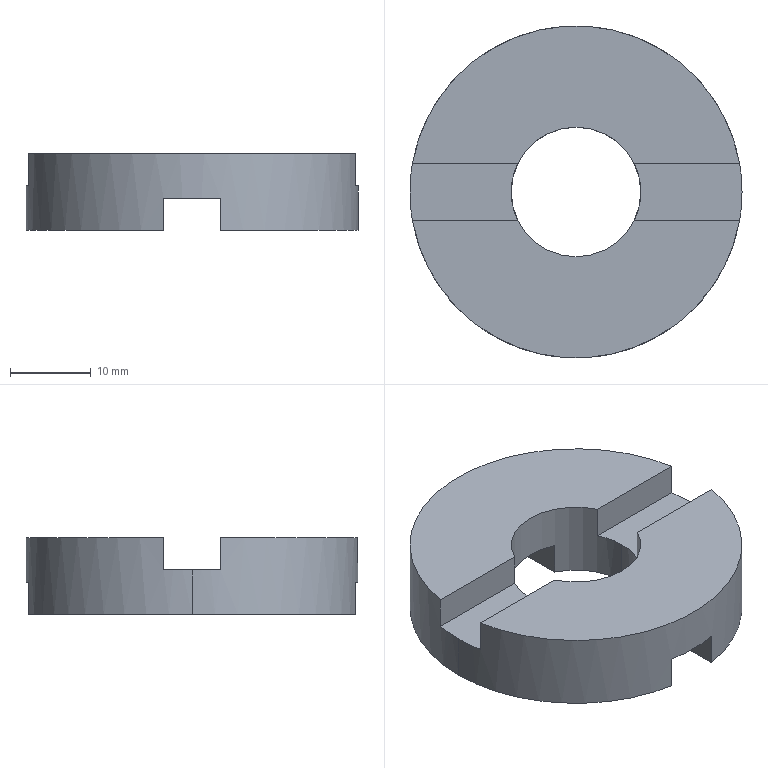Component | SolidWorks | ServoDriveMotorModule-1_MCOCGWK38_16_16-1_MCOCG_spacer38-1 | 1 solid | 20 faces | box 41 x 41 x 9.5 mm | volume 9214 mm3 | plane 16 | cylinder 4 | commonest cylinder face diameters 16 x2 41 x2 | material AISI 1045 Steel, cold drawn
build123d program:
from build123d import *

# Parameters (mm, degrees)
SKETCH1_W               = 9.5
SKETCH1_H               = 12.5
CUT_EXTRUDE1_DEPTH      = 20.5
CUT_EXTRUDE1_DEPTH_BACK = 20.5
SKETCH2_W               = 4
SKETCH2_H               = 7
CUT_EXTRUDE2_DEPTH      = 20.5
CUT_EXTRUDE2_DEPTH_BACK = 20.5
SKETCH3_W               = 4
SKETCH3_H               = 7


with BuildPart() as part:
    # Sketch1 → Revolve1 (revolve)
    with BuildSketch(Plane.XY, mode=Mode.PRIVATE) as revolve1_sk:
        with Locations((4.75, 14.25)):
            Rectangle(SKETCH1_W, SKETCH1_H)
    revolve(revolve1_sk.sketch.rotate(Axis((9.5, 0, 0), (-1, 0, 0)), 270), axis=Axis((9.5, 0, 0), (-1, 0, 0)))

    # Sketch2 → Cut-Extrude1 (cut, two sides: drawn at the far end of the back side and taken through both)
    with BuildSketch(Plane.XY.offset(-CUT_EXTRUDE1_DEPTH_BACK)):
        with Locations((2, 0)):
            Rectangle(SKETCH2_W, SKETCH2_H)
    extrude(amount=CUT_EXTRUDE1_DEPTH + CUT_EXTRUDE1_DEPTH_BACK, mode=Mode.SUBTRACT)

    # Sketch3 → Cut-Extrude2 (cut, two sides: drawn at the far end of the back side and taken through both)
    with BuildSketch(Plane(origin=(0, 0, 0), x_dir=(1, 0, 0), z_dir=(0, 1, 0)).offset(-CUT_EXTRUDE2_DEPTH_BACK)):
        with Locations((7.5, 0)):
            Rectangle(SKETCH3_W, SKETCH3_H)
    extrude(amount=CUT_EXTRUDE2_DEPTH + CUT_EXTRUDE2_DEPTH_BACK, mode=Mode.SUBTRACT)


solid = part.part

# Placed as in the assembly
solid = solid.moved(Location((0, 0, 101), (0, 90, 0)))
STEP:
#1=COLOUR_RGB('',0.7922,0.8196,0.9333);
#2=FILL_AREA_STYLE_COLOUR('',#1);
#3=FILL_AREA_STYLE('',(#2));
#4=SURFACE_STYLE_FILL_AREA(#3);
#5=SURFACE_SIDE_STYLE('',(#4));
#6=SURFACE_STYLE_USAGE(.BOTH.,#5);
#7=PRESENTATION_STYLE_ASSIGNMENT((#6));
#8=CARTESIAN_POINT('',(-0.315,0.,3.602));
#9=VERTEX_POINT('',#8);
#10=CARTESIAN_POINT('',(-0.1378,-0.2832,3.602));
#11=VERTEX_POINT('',#10);
#12=CARTESIAN_POINT('',(0.,0.,3.602));
#13=DIRECTION('',(0.,-0.,1.));
#14=DIRECTION('',(1.,0.,0.));
#15=AXIS2_PLACEMENT_3D('',#12,#13,#14);
#16=CIRCLE('',#15,0.315);
#17=EDGE_CURVE('',#9,#11,#16,.T.);
#18=ORIENTED_EDGE('',*,*,#17,.F.);
#19=CARTESIAN_POINT('',(-0.315,0.,3.819));
#20=VERTEX_POINT('',#19);
#21=CARTESIAN_POINT('',(-0.315,0.,3.602));
#22=DIRECTION('',(0.,-0.,1.));
#23=VECTOR('',#22,39.37);
#24=LINE('',#21,#23);
#25=EDGE_CURVE('',#9,#20,#24,.T.);
#26=ORIENTED_EDGE('',*,*,#25,.T.);
#27=CARTESIAN_POINT('',(-0.2832,-0.1378,3.819));
#28=VERTEX_POINT('',#27);
#29=CARTESIAN_POINT('',(0.,0.,3.819));
#30=DIRECTION('',(0.,-0.,1.));
#31=DIRECTION('',(-1.,-0.,0.));
#32=AXIS2_PLACEMENT_3D('',#29,#30,#31);
#33=CIRCLE('',#32,0.315);
#34=EDGE_CURVE('',#20,#28,#33,.T.);
#35=ORIENTED_EDGE('',*,*,#34,.T.);
#36=CARTESIAN_POINT('',(-0.2832,-0.1378,3.976));
#37=VERTEX_POINT('',#36);
#38=CARTESIAN_POINT('',(-0.2832,-0.1378,3.602));
#39=DIRECTION('',(0.,-0.,1.));
#40=VECTOR('',#39,39.37);
#41=LINE('',#38,#40);
#42=EDGE_CURVE('',#28,#37,#41,.T.);
#43=ORIENTED_EDGE('',*,*,#42,.T.);
#44=CARTESIAN_POINT('',(0.2832,-0.1378,3.976));
#45=VERTEX_POINT('',#44);
#46=CARTESIAN_POINT('',(0.,0.,3.976));
#47=DIRECTION('',(0.,-0.,1.));
#48=DIRECTION('',(1.,0.,0.));
#49=AXIS2_PLACEMENT_3D('',#46,#47,#48);
#50=CIRCLE('',#49,0.315);
#51=EDGE_CURVE('',#37,#45,#50,.T.);
#52=ORIENTED_EDGE('',*,*,#51,.T.);
#53=CARTESIAN_POINT('',(0.2832,-0.1378,3.819));
#54=VERTEX_POINT('',#53);
#55=CARTESIAN_POINT('',(0.2832,-0.1378,3.602));
#56=DIRECTION('',(-0.,0.,-1.));
#57=VECTOR('',#56,39.37);
#58=LINE('',#55,#57);
#59=EDGE_CURVE('',#45,#54,#58,.T.);
#60=ORIENTED_EDGE('',*,*,#59,.T.);
#61=CARTESIAN_POINT('',(0.315,0.,3.819));
#62=VERTEX_POINT('',#61);
#63=CARTESIAN_POINT('',(0.,0.,3.819));
#64=DIRECTION('',(0.,-0.,1.));
#65=DIRECTION('',(-1.,0.,0.));
#66=AXIS2_PLACEMENT_3D('',#63,#64,#65);
#67=CIRCLE('',#66,0.315);
#68=EDGE_CURVE('',#54,#62,#67,.T.);
#69=ORIENTED_EDGE('',*,*,#68,.T.);
#70=CARTESIAN_POINT('',(0.315,0.,3.602));
#71=VERTEX_POINT('',#70);
#72=CARTESIAN_POINT('',(0.315,0.,3.602));
#73=DIRECTION('',(0.,-0.,1.));
#74=VECTOR('',#73,39.37);
#75=LINE('',#72,#74);
#76=EDGE_CURVE('',#71,#62,#75,.T.);
#77=ORIENTED_EDGE('',*,*,#76,.F.);
#78=CARTESIAN_POINT('',(0.1378,-0.2832,3.602));
#79=VERTEX_POINT('',#78);
#80=CARTESIAN_POINT('',(0.,0.,3.602));
#81=DIRECTION('',(0.,-0.,1.));
#82=DIRECTION('',(1.,0.,0.));
#83=AXIS2_PLACEMENT_3D('',#80,#81,#82);
#84=CIRCLE('',#83,0.315);
#85=EDGE_CURVE('',#79,#71,#84,.T.);
#86=ORIENTED_EDGE('',*,*,#85,.F.);
#87=CARTESIAN_POINT('',(0.1378,-0.2832,3.76));
#88=VERTEX_POINT('',#87);
#89=CARTESIAN_POINT('',(0.1378,-0.2832,3.602));
#90=DIRECTION('',(0.,-0.,1.));
#91=VECTOR('',#90,39.37);
#92=LINE('',#89,#91);
#93=EDGE_CURVE('',#79,#88,#92,.T.);
#94=ORIENTED_EDGE('',*,*,#93,.T.);
#95=CARTESIAN_POINT('',(-0.1378,-0.2832,3.76));
#96=VERTEX_POINT('',#95);
#97=CARTESIAN_POINT('',(0.,0.,3.76));
#98=DIRECTION('',(-0.,0.,-1.));
#99=DIRECTION('',(1.,0.,0.));
#100=AXIS2_PLACEMENT_3D('',#97,#98,#99);
#101=CIRCLE('',#100,0.315);
#102=EDGE_CURVE('',#88,#96,#101,.T.);
#103=ORIENTED_EDGE('',*,*,#102,.T.);
#104=CARTESIAN_POINT('',(-0.1378,-0.2832,3.602));
#105=DIRECTION('',(-0.,0.,-1.));
#106=VECTOR('',#105,39.37);
#107=LINE('',#104,#106);
#108=EDGE_CURVE('',#96,#11,#107,.T.);
#109=ORIENTED_EDGE('',*,*,#108,.T.);
#110=EDGE_LOOP('',(#18,#26,#35,#43,#52,#60,#69,#77,#86,#94,#103,#109));
#111=FACE_OUTER_BOUND('',#110,.T.);
#112=CARTESIAN_POINT('',(0.,0.,3.602));
#113=DIRECTION('',(0.,-0.,1.));
#114=DIRECTION('',(1.,0.,0.));
#115=AXIS2_PLACEMENT_3D('',#112,#113,#114);
#116=CYLINDRICAL_SURFACE('',#115,0.315);
#117=ADVANCED_FACE('',(#111),#116,.F.);
#118=CARTESIAN_POINT('',(-0.1378,0.7952,3.602));
#119=VERTEX_POINT('',#118);
#120=CARTESIAN_POINT('',(-0.8071,-0.,3.602));
#121=VERTEX_POINT('',#120);
#122=CARTESIAN_POINT('',(0.,0.,3.602));
#123=DIRECTION('',(0.,-0.,1.));
#124=DIRECTION('',(1.,0.,0.));
#125=AXIS2_PLACEMENT_3D('',#122,#123,#124);
#126=CIRCLE('',#125,0.8071);
#127=EDGE_CURVE('',#119,#121,#126,.T.);
#128=ORIENTED_EDGE('',*,*,#127,.T.);
#129=CARTESIAN_POINT('',(-0.8071,-0.,3.819));
#130=VERTEX_POINT('',#129);
#131=CARTESIAN_POINT('',(-0.8071,-0.,3.602));
#132=DIRECTION('',(0.,-0.,1.));
#133=VECTOR('',#132,39.37);
#134=LINE('',#131,#133);
#135=EDGE_CURVE('',#121,#130,#134,.T.);
#136=ORIENTED_EDGE('',*,*,#135,.T.);
#137=CARTESIAN_POINT('',(-0.7952,0.1378,3.819));
#138=VERTEX_POINT('',#137);
#139=CARTESIAN_POINT('',(0.,0.,3.819));
#140=DIRECTION('',(-0.,0.,-1.));
#141=DIRECTION('',(-1.,-0.,0.));
#142=AXIS2_PLACEMENT_3D('',#139,#140,#141);
#143=CIRCLE('',#142,0.8071);
#144=EDGE_CURVE('',#130,#138,#143,.T.);
#145=ORIENTED_EDGE('',*,*,#144,.T.);
#146=CARTESIAN_POINT('',(-0.7952,0.1378,3.976));
#147=VERTEX_POINT('',#146);
#148=CARTESIAN_POINT('',(-0.7952,0.1378,3.602));
#149=DIRECTION('',(0.,-0.,1.));
#150=VECTOR('',#149,39.37);
#151=LINE('',#148,#150);
#152=EDGE_CURVE('',#138,#147,#151,.T.);
#153=ORIENTED_EDGE('',*,*,#152,.T.);
#154=CARTESIAN_POINT('',(0.7952,0.1378,3.976));
#155=VERTEX_POINT('',#154);
#156=CARTESIAN_POINT('',(0.,0.,3.976));
#157=DIRECTION('',(0.,-0.,1.));
#158=DIRECTION('',(1.,0.,0.));
#159=AXIS2_PLACEMENT_3D('',#156,#157,#158);
#160=CIRCLE('',#159,0.8071);
#161=EDGE_CURVE('',#155,#147,#160,.T.);
#162=ORIENTED_EDGE('',*,*,#161,.F.);
#163=CARTESIAN_POINT('',(0.7952,0.1378,3.819));
#164=VERTEX_POINT('',#163);
#165=CARTESIAN_POINT('',(0.7952,0.1378,3.602));
#166=DIRECTION('',(-0.,0.,-1.));
#167=VECTOR('',#166,39.37);
#168=LINE('',#165,#167);
#169=EDGE_CURVE('',#155,#164,#168,.T.);
#170=ORIENTED_EDGE('',*,*,#169,.T.);
#171=CARTESIAN_POINT('',(0.8071,0.,3.819));
#172=VERTEX_POINT('',#171);
#173=CARTESIAN_POINT('',(0.,0.,3.819));
#174=DIRECTION('',(-0.,0.,-1.));
#175=DIRECTION('',(-1.,-0.,0.));
#176=AXIS2_PLACEMENT_3D('',#173,#174,#175);
#177=CIRCLE('',#176,0.8071);
#178=EDGE_CURVE('',#164,#172,#177,.T.);
#179=ORIENTED_EDGE('',*,*,#178,.T.);
#180=CARTESIAN_POINT('',(0.8071,0.,3.602));
#181=VERTEX_POINT('',#180);
#182=CARTESIAN_POINT('',(0.8071,0.,3.602));
#183=DIRECTION('',(0.,-0.,1.));
#184=VECTOR('',#183,39.37);
#185=LINE('',#182,#184);
#186=EDGE_CURVE('',#181,#172,#185,.T.);
#187=ORIENTED_EDGE('',*,*,#186,.F.);
#188=CARTESIAN_POINT('',(0.1378,0.7952,3.602));
#189=VERTEX_POINT('',#188);
#190=CARTESIAN_POINT('',(0.,0.,3.602));
#191=DIRECTION('',(0.,-0.,1.));
#192=DIRECTION('',(1.,0.,0.));
#193=AXIS2_PLACEMENT_3D('',#190,#191,#192);
#194=CIRCLE('',#193,0.8071);
#195=EDGE_CURVE('',#181,#189,#194,.T.);
#196=ORIENTED_EDGE('',*,*,#195,.T.);
#197=CARTESIAN_POINT('',(0.1378,0.7952,3.76));
#198=VERTEX_POINT('',#197);
#199=CARTESIAN_POINT('',(0.1378,0.7952,3.602));
#200=DIRECTION('',(0.,-0.,1.));
#201=VECTOR('',#200,39.37);
#202=LINE('',#199,#201);
#203=EDGE_CURVE('',#189,#198,#202,.T.);
#204=ORIENTED_EDGE('',*,*,#203,.T.);
#205=CARTESIAN_POINT('',(-0.1378,0.7952,3.76));
#206=VERTEX_POINT('',#205);
#207=CARTESIAN_POINT('',(0.,0.,3.76));
#208=DIRECTION('',(0.,-0.,1.));
#209=DIRECTION('',(1.,0.,0.));
#210=AXIS2_PLACEMENT_3D('',#207,#208,#209);
#211=CIRCLE('',#210,0.8071);
#212=EDGE_CURVE('',#198,#206,#211,.T.);
#213=ORIENTED_EDGE('',*,*,#212,.T.);
#214=CARTESIAN_POINT('',(-0.1378,0.7952,3.602));
#215=DIRECTION('',(-0.,0.,-1.));
#216=VECTOR('',#215,39.37);
#217=LINE('',#214,#216);
#218=EDGE_CURVE('',#206,#119,#217,.T.);
#219=ORIENTED_EDGE('',*,*,#218,.T.);
#220=EDGE_LOOP('',(#128,#136,#145,#153,#162,#170,#179,#187,#196,#204,#213,#219));
#221=FACE_OUTER_BOUND('',#220,.T.);
#222=CARTESIAN_POINT('',(0.,0.,3.602));
#223=DIRECTION('',(0.,-0.,1.));
#224=DIRECTION('',(1.,0.,0.));
#225=AXIS2_PLACEMENT_3D('',#222,#223,#224);
#226=CYLINDRICAL_SURFACE('',#225,0.8071);
#227=ADVANCED_FACE('',(#221),#226,.T.);
#228=ORIENTED_EDGE('',*,*,#127,.F.);
#229=CARTESIAN_POINT('',(-0.1378,0.2832,3.602));
#230=VERTEX_POINT('',#229);
#231=CARTESIAN_POINT('',(-0.1378,0.315,3.602));
#232=DIRECTION('',(0.,-1.,-0.));
#233=VECTOR('',#232,39.37);
#234=LINE('',#231,#233);
#235=EDGE_CURVE('',#119,#230,#234,.T.);
#236=ORIENTED_EDGE('',*,*,#235,.T.);
#237=CARTESIAN_POINT('',(0.,0.,3.602));
#238=DIRECTION('',(0.,-0.,1.));
#239=DIRECTION('',(1.,0.,0.));
#240=AXIS2_PLACEMENT_3D('',#237,#238,#239);
#241=CIRCLE('',#240,0.315);
#242=EDGE_CURVE('',#230,#9,#241,.T.);
#243=ORIENTED_EDGE('',*,*,#242,.T.);
#244=ORIENTED_EDGE('',*,*,#17,.T.);
#245=CARTESIAN_POINT('',(-0.1378,-0.7952,3.602));
#246=VERTEX_POINT('',#245);
#247=CARTESIAN_POINT('',(-0.1378,0.315,3.602));
#248=DIRECTION('',(0.,-1.,-0.));
#249=VECTOR('',#248,39.37);
#250=LINE('',#247,#249);
#251=EDGE_CURVE('',#11,#246,#250,.T.);
#252=ORIENTED_EDGE('',*,*,#251,.T.);
#253=CARTESIAN_POINT('',(0.,0.,3.602));
#254=DIRECTION('',(0.,-0.,1.));
#255=DIRECTION('',(1.,0.,0.));
#256=AXIS2_PLACEMENT_3D('',#253,#254,#255);
#257=CIRCLE('',#256,0.8071);
#258=EDGE_CURVE('',#121,#246,#257,.T.);
#259=ORIENTED_EDGE('',*,*,#258,.F.);
#260=EDGE_LOOP('',(#228,#236,#243,#244,#252,#259));
#261=FACE_OUTER_BOUND('',#260,.T.);
#262=CARTESIAN_POINT('',(0.,0.315,3.602));
#263=DIRECTION('',(0.,-0.,1.));
#264=DIRECTION('',(1.,0.,-0.));
#265=AXIS2_PLACEMENT_3D('',#262,#263,#264);
#266=PLANE('',#265);
#267=ADVANCED_FACE('',(#261),#266,.F.);
#268=ORIENTED_EDGE('',*,*,#161,.T.);
#269=CARTESIAN_POINT('',(-0.2832,0.1378,3.976));
#270=VERTEX_POINT('',#269);
#271=CARTESIAN_POINT('',(-0.8071,0.1378,3.976));
#272=DIRECTION('',(1.,0.,-0.));
#273=VECTOR('',#272,39.37);
#274=LINE('',#271,#273);
#275=EDGE_CURVE('',#147,#270,#274,.T.);
#276=ORIENTED_EDGE('',*,*,#275,.T.);
#277=CARTESIAN_POINT('',(0.2832,0.1378,3.976));
#278=VERTEX_POINT('',#277);
#279=CARTESIAN_POINT('',(0.,0.,3.976));
#280=DIRECTION('',(0.,-0.,1.));
#281=DIRECTION('',(1.,0.,0.));
#282=AXIS2_PLACEMENT_3D('',#279,#280,#281);
#283=CIRCLE('',#282,0.315);
#284=EDGE_CURVE('',#278,#270,#283,.T.);
#285=ORIENTED_EDGE('',*,*,#284,.F.);
#286=CARTESIAN_POINT('',(-0.8071,0.1378,3.976));
#287=DIRECTION('',(1.,0.,-0.));
#288=VECTOR('',#287,39.37);
#289=LINE('',#286,#288);
#290=EDGE_CURVE('',#278,#155,#289,.T.);
#291=ORIENTED_EDGE('',*,*,#290,.T.);
#292=EDGE_LOOP('',(#268,#276,#285,#291));
#293=FACE_OUTER_BOUND('',#292,.T.);
#294=CARTESIAN_POINT('',(0.,0.8071,3.976));
#295=DIRECTION('',(-0.,0.,-1.));
#296=DIRECTION('',(-1.,-0.,0.));
#297=AXIS2_PLACEMENT_3D('',#294,#295,#296);
#298=PLANE('',#297);
#299=ADVANCED_FACE('',(#293),#298,.F.);
#300=ORIENTED_EDGE('',*,*,#135,.F.);
#301=ORIENTED_EDGE('',*,*,#258,.T.);
#302=CARTESIAN_POINT('',(-0.1378,-0.7952,3.76));
#303=VERTEX_POINT('',#302);
#304=CARTESIAN_POINT('',(-0.1378,-0.7952,3.602));
#305=DIRECTION('',(0.,-0.,1.));
#306=VECTOR('',#305,39.37);
#307=LINE('',#304,#306);
#308=EDGE_CURVE('',#246,#303,#307,.T.);
#309=ORIENTED_EDGE('',*,*,#308,.T.);
#310=CARTESIAN_POINT('',(0.1378,-0.7952,3.76));
#311=VERTEX_POINT('',#310);
#312=CARTESIAN_POINT('',(0.,0.,3.76));
#313=DIRECTION('',(0.,-0.,1.));
#314=DIRECTION('',(1.,0.,0.));
#315=AXIS2_PLACEMENT_3D('',#312,#313,#314);
#316=CIRCLE('',#315,0.8071);
#317=EDGE_CURVE('',#303,#311,#316,.T.);
#318=ORIENTED_EDGE('',*,*,#317,.T.);
#319=CARTESIAN_POINT('',(0.1378,-0.7952,3.602));
#320=VERTEX_POINT('',#319);
#321=CARTESIAN_POINT('',(0.1378,-0.7952,3.602));
#322=DIRECTION('',(-0.,0.,-1.));
#323=VECTOR('',#322,39.37);
#324=LINE('',#321,#323);
#325=EDGE_CURVE('',#311,#320,#324,.T.);
#326=ORIENTED_EDGE('',*,*,#325,.T.);
#327=CARTESIAN_POINT('',(0.,0.,3.602));
#328=DIRECTION('',(0.,-0.,1.));
#329=DIRECTION('',(1.,0.,0.));
#330=AXIS2_PLACEMENT_3D('',#327,#328,#329);
#331=CIRCLE('',#330,0.8071);
#332=EDGE_CURVE('',#320,#181,#331,.T.);
#333=ORIENTED_EDGE('',*,*,#332,.T.);
#334=ORIENTED_EDGE('',*,*,#186,.T.);
#335=CARTESIAN_POINT('',(0.7952,-0.1378,3.819));
#336=VERTEX_POINT('',#335);
#337=CARTESIAN_POINT('',(0.,0.,3.819));
#338=DIRECTION('',(-0.,0.,-1.));
#339=DIRECTION('',(-1.,-0.,0.));
#340=AXIS2_PLACEMENT_3D('',#337,#338,#339);
#341=CIRCLE('',#340,0.8071);
#342=EDGE_CURVE('',#172,#336,#341,.T.);
#343=ORIENTED_EDGE('',*,*,#342,.T.);
#344=CARTESIAN_POINT('',(0.7952,-0.1378,3.976));
#345=VERTEX_POINT('',#344);
#346=CARTESIAN_POINT('',(0.7952,-0.1378,3.602));
#347=DIRECTION('',(0.,-0.,1.));
#348=VECTOR('',#347,39.37);
#349=LINE('',#346,#348);
#350=EDGE_CURVE('',#336,#345,#349,.T.);
#351=ORIENTED_EDGE('',*,*,#350,.T.);
#352=CARTESIAN_POINT('',(-0.7952,-0.1378,3.976));
#353=VERTEX_POINT('',#352);
#354=CARTESIAN_POINT('',(0.,0.,3.976));
#355=DIRECTION('',(0.,-0.,1.));
#356=DIRECTION('',(1.,0.,0.));
#357=AXIS2_PLACEMENT_3D('',#354,#355,#356);
#358=CIRCLE('',#357,0.8071);
#359=EDGE_CURVE('',#353,#345,#358,.T.);
#360=ORIENTED_EDGE('',*,*,#359,.F.);
#361=CARTESIAN_POINT('',(-0.7952,-0.1378,3.819));
#362=VERTEX_POINT('',#361);
#363=CARTESIAN_POINT('',(-0.7952,-0.1378,3.602));
#364=DIRECTION('',(-0.,0.,-1.));
#365=VECTOR('',#364,39.37);
#366=LINE('',#363,#365);
#367=EDGE_CURVE('',#353,#362,#366,.T.);
#368=ORIENTED_EDGE('',*,*,#367,.T.);
#369=CARTESIAN_POINT('',(0.,0.,3.819));
#370=DIRECTION('',(-0.,0.,-1.));
#371=DIRECTION('',(-1.,-0.,0.));
#372=AXIS2_PLACEMENT_3D('',#369,#370,#371);
#373=CIRCLE('',#372,0.8071);
#374=EDGE_CURVE('',#362,#130,#373,.T.);
#375=ORIENTED_EDGE('',*,*,#374,.T.);
#376=EDGE_LOOP('',(#300,#301,#309,#318,#326,#333,#334,#343,#351,#360,#368,#375));
#377=FACE_OUTER_BOUND('',#376,.T.);
#378=CARTESIAN_POINT('',(0.,0.,3.602));
#379=DIRECTION('',(0.,-0.,1.));
#380=DIRECTION('',(1.,0.,0.));
#381=AXIS2_PLACEMENT_3D('',#378,#379,#380);
#382=CYLINDRICAL_SURFACE('',#381,0.8071);
#383=ADVANCED_FACE('',(#377),#382,.T.);
#384=ORIENTED_EDGE('',*,*,#359,.T.);
#385=CARTESIAN_POINT('',(-0.8071,-0.1378,3.976));
#386=DIRECTION('',(1.,0.,-0.));
#387=VECTOR('',#386,39.37);
#388=LINE('',#385,#387);
#389=EDGE_CURVE('',#45,#345,#388,.T.);
#390=ORIENTED_EDGE('',*,*,#389,.F.);
#391=ORIENTED_EDGE('',*,*,#51,.F.);
#392=CARTESIAN_POINT('',(-0.8071,-0.1378,3.976));
#393=DIRECTION('',(1.,0.,-0.));
#394=VECTOR('',#393,39.37);
#395=LINE('',#392,#394);
#396=EDGE_CURVE('',#353,#37,#395,.T.);
#397=ORIENTED_EDGE('',*,*,#396,.F.);
#398=EDGE_LOOP('',(#384,#390,#391,#397));
#399=FACE_OUTER_BOUND('',#398,.T.);
#400=CARTESIAN_POINT('',(0.,0.8071,3.976));
#401=DIRECTION('',(-0.,0.,-1.));
#402=DIRECTION('',(-1.,-0.,0.));
#403=AXIS2_PLACEMENT_3D('',#400,#401,#402);
#404=PLANE('',#403);
#405=ADVANCED_FACE('',(#399),#404,.F.);
#406=ORIENTED_EDGE('',*,*,#25,.F.);
#407=ORIENTED_EDGE('',*,*,#242,.F.);
#408=CARTESIAN_POINT('',(-0.1378,0.2832,3.76));
#409=VERTEX_POINT('',#408);
#410=CARTESIAN_POINT('',(-0.1378,0.2832,3.602));
#411=DIRECTION('',(0.,-0.,1.));
#412=VECTOR('',#411,39.37);
#413=LINE('',#410,#412);
#414=EDGE_CURVE('',#230,#409,#413,.T.);
#415=ORIENTED_EDGE('',*,*,#414,.T.);
#416=CARTESIAN_POINT('',(0.1378,0.2832,3.76));
#417=VERTEX_POINT('',#416);
#418=CARTESIAN_POINT('',(0.,0.,3.76));
#419=DIRECTION('',(-0.,0.,-1.));
#420=DIRECTION('',(1.,0.,0.));
#421=AXIS2_PLACEMENT_3D('',#418,#419,#420);
#422=CIRCLE('',#421,0.315);
#423=EDGE_CURVE('',#409,#417,#422,.T.);
#424=ORIENTED_EDGE('',*,*,#423,.T.);
#425=CARTESIAN_POINT('',(0.1378,0.2832,3.602));
#426=VERTEX_POINT('',#425);
#427=CARTESIAN_POINT('',(0.1378,0.2832,3.602));
#428=DIRECTION('',(-0.,0.,-1.));
#429=VECTOR('',#428,39.37);
#430=LINE('',#427,#429);
#431=EDGE_CURVE('',#417,#426,#430,.T.);
#432=ORIENTED_EDGE('',*,*,#431,.T.);
#433=CARTESIAN_POINT('',(0.,0.,3.602));
#434=DIRECTION('',(0.,-0.,1.));
#435=DIRECTION('',(1.,0.,0.));
#436=AXIS2_PLACEMENT_3D('',#433,#434,#435);
#437=CIRCLE('',#436,0.315);
#438=EDGE_CURVE('',#71,#426,#437,.T.);
#439=ORIENTED_EDGE('',*,*,#438,.F.);
#440=ORIENTED_EDGE('',*,*,#76,.T.);
#441=CARTESIAN_POINT('',(0.2832,0.1378,3.819));
#442=VERTEX_POINT('',#441);
#443=CARTESIAN_POINT('',(0.,0.,3.819));
#444=DIRECTION('',(0.,-0.,1.));
#445=DIRECTION('',(-1.,-0.,0.));
#446=AXIS2_PLACEMENT_3D('',#443,#444,#445);
#447=CIRCLE('',#446,0.315);
#448=EDGE_CURVE('',#62,#442,#447,.T.);
#449=ORIENTED_EDGE('',*,*,#448,.T.);
#450=CARTESIAN_POINT('',(0.2832,0.1378,3.602));
#451=DIRECTION('',(0.,-0.,1.));
#452=VECTOR('',#451,39.37);
#453=LINE('',#450,#452);
#454=EDGE_CURVE('',#442,#278,#453,.T.);
#455=ORIENTED_EDGE('',*,*,#454,.T.);
#456=ORIENTED_EDGE('',*,*,#284,.T.);
#457=CARTESIAN_POINT('',(-0.2832,0.1378,3.819));
#458=VERTEX_POINT('',#457);
#459=CARTESIAN_POINT('',(-0.2832,0.1378,3.602));
#460=DIRECTION('',(-0.,0.,-1.));
#461=VECTOR('',#460,39.37);
#462=LINE('',#459,#461);
#463=EDGE_CURVE('',#270,#458,#462,.T.);
#464=ORIENTED_EDGE('',*,*,#463,.T.);
#465=CARTESIAN_POINT('',(0.,0.,3.819));
#466=DIRECTION('',(0.,-0.,1.));
#467=DIRECTION('',(-1.,-0.,0.));
#468=AXIS2_PLACEMENT_3D('',#465,#466,#467);
#469=CIRCLE('',#468,0.315);
#470=EDGE_CURVE('',#458,#20,#469,.T.);
#471=ORIENTED_EDGE('',*,*,#470,.T.);
#472=EDGE_LOOP('',(#406,#407,#415,#424,#432,#439,#440,#449,#455,#456,#464,#471));
#473=FACE_OUTER_BOUND('',#472,.T.);
#474=CARTESIAN_POINT('',(0.,0.,3.602));
#475=DIRECTION('',(0.,-0.,1.));
#476=DIRECTION('',(1.,0.,0.));
#477=AXIS2_PLACEMENT_3D('',#474,#475,#476);
#478=CYLINDRICAL_SURFACE('',#477,0.315);
#479=ADVANCED_FACE('',(#473),#478,.F.);
#480=ORIENTED_EDGE('',*,*,#332,.F.);
#481=CARTESIAN_POINT('',(0.1378,0.315,3.602));
#482=DIRECTION('',(-0.,1.,0.));
#483=VECTOR('',#482,39.37);
#484=LINE('',#481,#483);
#485=EDGE_CURVE('',#320,#79,#484,.T.);
#486=ORIENTED_EDGE('',*,*,#485,.T.);
#487=ORIENTED_EDGE('',*,*,#85,.T.);
#488=ORIENTED_EDGE('',*,*,#438,.T.);
#489=CARTESIAN_POINT('',(0.1378,0.315,3.602));
#490=DIRECTION('',(-0.,1.,0.));
#491=VECTOR('',#490,39.37);
#492=LINE('',#489,#491);
#493=EDGE_CURVE('',#426,#189,#492,.T.);
#494=ORIENTED_EDGE('',*,*,#493,.T.);
#495=ORIENTED_EDGE('',*,*,#195,.F.);
#496=EDGE_LOOP('',(#480,#486,#487,#488,#494,#495));
#497=FACE_OUTER_BOUND('',#496,.T.);
#498=CARTESIAN_POINT('',(0.,0.315,3.602));
#499=DIRECTION('',(0.,-0.,1.));
#500=DIRECTION('',(1.,0.,-0.));
#501=AXIS2_PLACEMENT_3D('',#498,#499,#500);
#502=PLANE('',#501);
#503=ADVANCED_FACE('',(#497),#502,.F.);
#504=ORIENTED_EDGE('',*,*,#396,.T.);
#505=ORIENTED_EDGE('',*,*,#42,.F.);
#506=CARTESIAN_POINT('',(-0.8071,-0.1378,3.819));
#507=DIRECTION('',(1.,0.,-0.));
#508=VECTOR('',#507,39.37);
#509=LINE('',#506,#508);
#510=EDGE_CURVE('',#362,#28,#509,.T.);
#511=ORIENTED_EDGE('',*,*,#510,.F.);
#512=ORIENTED_EDGE('',*,*,#367,.F.);
#513=EDGE_LOOP('',(#504,#505,#511,#512));
#514=FACE_OUTER_BOUND('',#513,.T.);
#515=CARTESIAN_POINT('',(-0.8071,-0.1378,3.976));
#516=DIRECTION('',(0.,-1.,-0.));
#517=DIRECTION('',(-1.,-0.,0.));
#518=AXIS2_PLACEMENT_3D('',#515,#516,#517);
#519=PLANE('',#518);
#520=ADVANCED_FACE('',(#514),#519,.F.);
#521=ORIENTED_EDGE('',*,*,#374,.F.);
#522=ORIENTED_EDGE('',*,*,#510,.T.);
#523=ORIENTED_EDGE('',*,*,#34,.F.);
#524=ORIENTED_EDGE('',*,*,#470,.F.);
#525=CARTESIAN_POINT('',(-0.8071,0.1378,3.819));
#526=DIRECTION('',(1.,0.,-0.));
#527=VECTOR('',#526,39.37);
#528=LINE('',#525,#527);
#529=EDGE_CURVE('',#138,#458,#528,.T.);
#530=ORIENTED_EDGE('',*,*,#529,.F.);
#531=ORIENTED_EDGE('',*,*,#144,.F.);
#532=EDGE_LOOP('',(#521,#522,#523,#524,#530,#531));
#533=FACE_OUTER_BOUND('',#532,.T.);
#534=CARTESIAN_POINT('',(-0.8071,-0.1378,3.819));
#535=DIRECTION('',(-0.,0.,-1.));
#536=DIRECTION('',(-1.,-0.,0.));
#537=AXIS2_PLACEMENT_3D('',#534,#535,#536);
#538=PLANE('',#537);
#539=ADVANCED_FACE('',(#533),#538,.F.);
#540=ORIENTED_EDGE('',*,*,#529,.T.);
#541=ORIENTED_EDGE('',*,*,#463,.F.);
#542=ORIENTED_EDGE('',*,*,#275,.F.);
#543=ORIENTED_EDGE('',*,*,#152,.F.);
#544=EDGE_LOOP('',(#540,#541,#542,#543));
#545=FACE_OUTER_BOUND('',#544,.T.);
#546=CARTESIAN_POINT('',(-0.8071,0.1378,3.819));
#547=DIRECTION('',(-0.,1.,0.));
#548=DIRECTION('',(1.,0.,-0.));
#549=AXIS2_PLACEMENT_3D('',#546,#547,#548);
#550=PLANE('',#549);
#551=ADVANCED_FACE('',(#545),#550,.F.);
#552=ORIENTED_EDGE('',*,*,#290,.F.);
#553=ORIENTED_EDGE('',*,*,#454,.F.);
#554=CARTESIAN_POINT('',(-0.8071,0.1378,3.819));
#555=DIRECTION('',(1.,0.,-0.));
#556=VECTOR('',#555,39.37);
#557=LINE('',#554,#556);
#558=EDGE_CURVE('',#442,#164,#557,.T.);
#559=ORIENTED_EDGE('',*,*,#558,.T.);
#560=ORIENTED_EDGE('',*,*,#169,.F.);
#561=EDGE_LOOP('',(#552,#553,#559,#560));
#562=FACE_OUTER_BOUND('',#561,.T.);
#563=CARTESIAN_POINT('',(-0.8071,0.1378,3.819));
#564=DIRECTION('',(-0.,1.,0.));
#565=DIRECTION('',(1.,0.,-0.));
#566=AXIS2_PLACEMENT_3D('',#563,#564,#565);
#567=PLANE('',#566);
#568=ADVANCED_FACE('',(#562),#567,.F.);
#569=ORIENTED_EDGE('',*,*,#558,.F.);
#570=ORIENTED_EDGE('',*,*,#448,.F.);
#571=ORIENTED_EDGE('',*,*,#68,.F.);
#572=CARTESIAN_POINT('',(-0.8071,-0.1378,3.819));
#573=DIRECTION('',(1.,0.,-0.));
#574=VECTOR('',#573,39.37);
#575=LINE('',#572,#574);
#576=EDGE_CURVE('',#54,#336,#575,.T.);
#577=ORIENTED_EDGE('',*,*,#576,.T.);
#578=ORIENTED_EDGE('',*,*,#342,.F.);
#579=ORIENTED_EDGE('',*,*,#178,.F.);
#580=EDGE_LOOP('',(#569,#570,#571,#577,#578,#579));
#581=FACE_OUTER_BOUND('',#580,.T.);
#582=CARTESIAN_POINT('',(-0.8071,-0.1378,3.819));
#583=DIRECTION('',(-0.,0.,-1.));
#584=DIRECTION('',(-1.,-0.,0.));
#585=AXIS2_PLACEMENT_3D('',#582,#583,#584);
#586=PLANE('',#585);
#587=ADVANCED_FACE('',(#581),#586,.F.);
#588=ORIENTED_EDGE('',*,*,#576,.F.);
#589=ORIENTED_EDGE('',*,*,#59,.F.);
#590=ORIENTED_EDGE('',*,*,#389,.T.);
#591=ORIENTED_EDGE('',*,*,#350,.F.);
#592=EDGE_LOOP('',(#588,#589,#590,#591));
#593=FACE_OUTER_BOUND('',#592,.T.);
#594=CARTESIAN_POINT('',(-0.8071,-0.1378,3.976));
#595=DIRECTION('',(0.,-1.,-0.));
#596=DIRECTION('',(-1.,-0.,0.));
#597=AXIS2_PLACEMENT_3D('',#594,#595,#596);
#598=PLANE('',#597);
#599=ADVANCED_FACE('',(#593),#598,.F.);
#600=CARTESIAN_POINT('',(-0.1378,-0.8071,3.76));
#601=DIRECTION('',(-0.,1.,0.));
#602=VECTOR('',#601,39.37);
#603=LINE('',#600,#602);
#604=EDGE_CURVE('',#409,#206,#603,.T.);
#605=ORIENTED_EDGE('',*,*,#604,.F.);
#606=ORIENTED_EDGE('',*,*,#414,.F.);
#607=ORIENTED_EDGE('',*,*,#235,.F.);
#608=ORIENTED_EDGE('',*,*,#218,.F.);
#609=EDGE_LOOP('',(#605,#606,#607,#608));
#610=FACE_OUTER_BOUND('',#609,.T.);
#611=CARTESIAN_POINT('',(-0.1378,-0.8071,3.602));
#612=DIRECTION('',(-1.,-0.,0.));
#613=DIRECTION('',(0.,-0.,1.));
#614=AXIS2_PLACEMENT_3D('',#611,#612,#613);
#615=PLANE('',#614);
#616=ADVANCED_FACE('',(#610),#615,.F.);
#617=ORIENTED_EDGE('',*,*,#493,.F.);
#618=ORIENTED_EDGE('',*,*,#431,.F.);
#619=CARTESIAN_POINT('',(0.1378,-0.8071,3.76));
#620=DIRECTION('',(-0.,1.,0.));
#621=VECTOR('',#620,39.37);
#622=LINE('',#619,#621);
#623=EDGE_CURVE('',#417,#198,#622,.T.);
#624=ORIENTED_EDGE('',*,*,#623,.T.);
#625=ORIENTED_EDGE('',*,*,#203,.F.);
#626=EDGE_LOOP('',(#617,#618,#624,#625));
#627=FACE_OUTER_BOUND('',#626,.T.);
#628=CARTESIAN_POINT('',(0.1378,-0.8071,3.76));
#629=DIRECTION('',(1.,0.,-0.));
#630=DIRECTION('',(-0.,0.,-1.));
#631=AXIS2_PLACEMENT_3D('',#628,#629,#630);
#632=PLANE('',#631);
#633=ADVANCED_FACE('',(#627),#632,.F.);
#634=ORIENTED_EDGE('',*,*,#623,.F.);
#635=ORIENTED_EDGE('',*,*,#423,.F.);
#636=ORIENTED_EDGE('',*,*,#604,.T.);
#637=ORIENTED_EDGE('',*,*,#212,.F.);
#638=EDGE_LOOP('',(#634,#635,#636,#637));
#639=FACE_OUTER_BOUND('',#638,.T.);
#640=CARTESIAN_POINT('',(-0.1378,-0.8071,3.76));
#641=DIRECTION('',(0.,-0.,1.));
#642=DIRECTION('',(1.,0.,-0.));
#643=AXIS2_PLACEMENT_3D('',#640,#641,#642);
#644=PLANE('',#643);
#645=ADVANCED_FACE('',(#639),#644,.F.);
#646=CARTESIAN_POINT('',(-0.1378,-0.8071,3.76));
#647=DIRECTION('',(-0.,1.,0.));
#648=VECTOR('',#647,39.37);
#649=LINE('',#646,#648);
#650=EDGE_CURVE('',#303,#96,#649,.T.);
#651=ORIENTED_EDGE('',*,*,#650,.T.);
#652=ORIENTED_EDGE('',*,*,#102,.F.);
#653=CARTESIAN_POINT('',(0.1378,-0.8071,3.76));
#654=DIRECTION('',(-0.,1.,0.));
#655=VECTOR('',#654,39.37);
#656=LINE('',#653,#655);
#657=EDGE_CURVE('',#311,#88,#656,.T.);
#658=ORIENTED_EDGE('',*,*,#657,.F.);
#659=ORIENTED_EDGE('',*,*,#317,.F.);
#660=EDGE_LOOP('',(#651,#652,#658,#659));
#661=FACE_OUTER_BOUND('',#660,.T.);
#662=CARTESIAN_POINT('',(-0.1378,-0.8071,3.76));
#663=DIRECTION('',(0.,-0.,1.));
#664=DIRECTION('',(1.,0.,-0.));
#665=AXIS2_PLACEMENT_3D('',#662,#663,#664);
#666=PLANE('',#665);
#667=ADVANCED_FACE('',(#661),#666,.F.);
#668=ORIENTED_EDGE('',*,*,#251,.F.);
#669=ORIENTED_EDGE('',*,*,#108,.F.);
#670=ORIENTED_EDGE('',*,*,#650,.F.);
#671=ORIENTED_EDGE('',*,*,#308,.F.);
#672=EDGE_LOOP('',(#668,#669,#670,#671));
#673=FACE_OUTER_BOUND('',#672,.T.);
#674=CARTESIAN_POINT('',(-0.1378,-0.8071,3.602));
#675=DIRECTION('',(-1.,-0.,0.));
#676=DIRECTION('',(0.,-0.,1.));
#677=AXIS2_PLACEMENT_3D('',#674,#675,#676);
#678=PLANE('',#677);
#679=ADVANCED_FACE('',(#673),#678,.F.);
#680=ORIENTED_EDGE('',*,*,#657,.T.);
#681=ORIENTED_EDGE('',*,*,#93,.F.);
#682=ORIENTED_EDGE('',*,*,#485,.F.);
#683=ORIENTED_EDGE('',*,*,#325,.F.);
#684=EDGE_LOOP('',(#680,#681,#682,#683));
#685=FACE_OUTER_BOUND('',#684,.T.);
#686=CARTESIAN_POINT('',(0.1378,-0.8071,3.76));
#687=DIRECTION('',(1.,0.,-0.));
#688=DIRECTION('',(-0.,0.,-1.));
#689=AXIS2_PLACEMENT_3D('',#686,#687,#688);
#690=PLANE('',#689);
#691=ADVANCED_FACE('',(#685),#690,.F.);
#692=CLOSED_SHELL('',(#117,#227,#267,#299,#383,#405,#479,#503,#520,#539,#551,#568,#587,#599,#616,#633,#645,#667,#679,#691));
#693=MANIFOLD_SOLID_BREP('',#692);
#694=STYLED_ITEM('',(#7),#693);
#695=(LENGTH_UNIT()NAMED_UNIT(*)SI_UNIT($,.METRE.));
#696=LENGTH_MEASURE_WITH_UNIT(LENGTH_MEASURE(0.0254),#695);
#697=DIMENSIONAL_EXPONENTS(1.,0.,0.,0.,0.,0.,0.);
#698=(CONVERSION_BASED_UNIT('',#696)LENGTH_UNIT()NAMED_UNIT(#697));
#699=UNCERTAINTY_MEASURE_WITH_UNIT(LENGTH_MEASURE(0.00001),#698,'','');
#700=(NAMED_UNIT(*)PLANE_ANGLE_UNIT()SI_UNIT($,.RADIAN.));
#701=(NAMED_UNIT(*)SI_UNIT($,.STERADIAN.)SOLID_ANGLE_UNIT());
#702=(GEOMETRIC_REPRESENTATION_CONTEXT(3)GLOBAL_UNCERTAINTY_ASSIGNED_CONTEXT((#699))GLOBAL_UNIT_ASSIGNED_CONTEXT((#698,#700,#701))REPRESENTATION_CONTEXT('',''));
#703=MECHANICAL_DESIGN_GEOMETRIC_PRESENTATION_REPRESENTATION('',(#694),#702);
#704=CARTESIAN_POINT('',(0.,0.,0.));
#705=DIRECTION('',(0.,0.,1.));
#706=DIRECTION('',(1.,0.,0.));
#707=AXIS2_PLACEMENT_3D('',#704,#705,#706);
#708=(LENGTH_UNIT()NAMED_UNIT(*)SI_UNIT($,.METRE.));
#709=LENGTH_MEASURE_WITH_UNIT(LENGTH_MEASURE(0.0254),#708);
#710=DIMENSIONAL_EXPONENTS(1.,0.,0.,0.,0.,0.,0.);
#711=(CONVERSION_BASED_UNIT('',#709)LENGTH_UNIT()NAMED_UNIT(#710));
#712=UNCERTAINTY_MEASURE_WITH_UNIT(LENGTH_MEASURE(0.00001),#711,'','');
#713=(NAMED_UNIT(*)PLANE_ANGLE_UNIT()SI_UNIT($,.RADIAN.));
#714=(NAMED_UNIT(*)SI_UNIT($,.STERADIAN.)SOLID_ANGLE_UNIT());
#715=(GEOMETRIC_REPRESENTATION_CONTEXT(3)GLOBAL_UNCERTAINTY_ASSIGNED_CONTEXT((#712))GLOBAL_UNIT_ASSIGNED_CONTEXT((#711,#713,#714))REPRESENTATION_CONTEXT('',''));
#716=ADVANCED_BREP_SHAPE_REPRESENTATION('',(#693,#707),#715);
#717=PRESENTATION_LAYER_ASSIGNMENT('','',(#694));